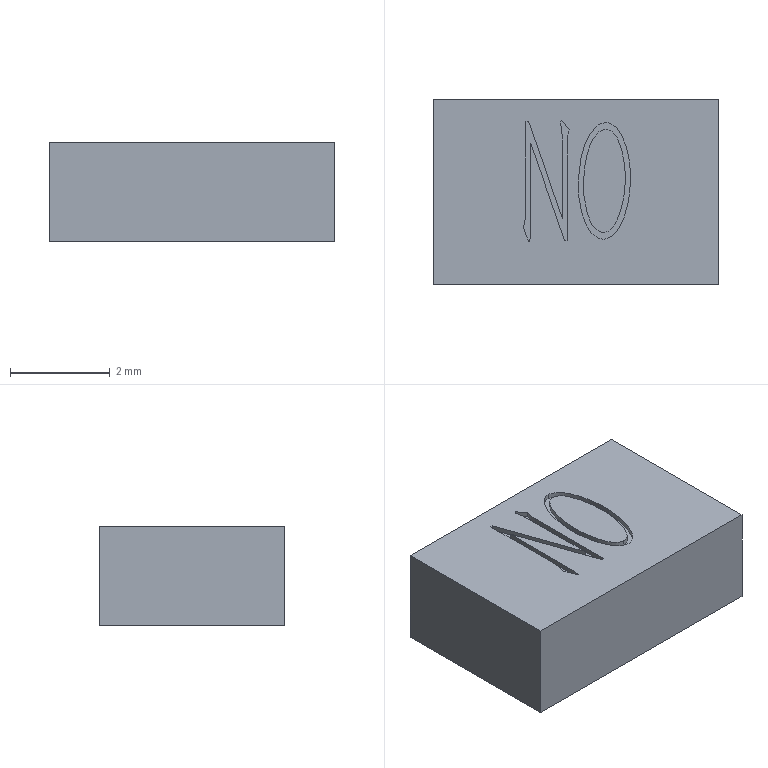Component | SolidWorks | Button1-1 | 1 solid | 33 faces | box 5.7 x 3.7 x 2 mm | volume 42 mm3 | plane 21 | spline 12
build123d program:
from build123d import *

# Parameters (mm, degrees)
SKETCH1_W           = 5.7
SKETCH1_H           = 3.7
BOSS_EXTRUDE1_DEPTH = 2
CUT_EXTRUDE1_DEPTH  = 0.1


with BuildPart() as part:
    # Sketch1 → Boss-Extrude1 (new body)
    with BuildSketch(Plane.XY):
        with Locations((2.85, 1.85)):
            Rectangle(SKETCH1_W, SKETCH1_H)
    extrude(amount=BOSS_EXTRUDE1_DEPTH)

    # Sketch2 → Cut-Extrude1 (cut)
    # profile 1 of 2: a face of its own
    with BuildSketch(Plane.XY.offset(2)):
        with BuildLine():
            Line((2.531, 3.25), (2.564, 3.282))
            Line((2.564, 3.282), (2.718, 3.092))
            add(Edge.make_bspline(
                [(2.718, 3.092), (2.715, 3.08), (2.708, 3.058), (2.697, 3.03), (2.691, 3.007), (2.687, 2.985), (2.683, 2.959), (2.679, 2.921), (2.676, 2.877), (2.675, 2.844), (2.675, 2.83)],
                knots=[0, 0, 0, 0, 1.084, 2.098, 2.644, 3.294, 4.083, 4.997, 6.707, 8, 8, 8, 8], degree=3))
            Line((2.675, 2.83), (2.675, 0.8842))
            Line((2.675, 0.8842), (2.621, 0.8842))
            Line((2.621, 0.8842), (1.945, 2.812))
            Line((1.945, 2.812), (1.945, 1.176))
            add(Edge.make_bspline(
                [(1.945, 1.176), (1.945, 1.162), (1.945, 1.133), (1.944, 1.087), (1.941, 1.036), (1.938, 0.9825), (1.935, 0.9341), (1.93, 0.8958), (1.927, 0.8739), (1.92, 0.8578), (1.905, 0.864), (1.894, 0.8769), (1.881, 0.9018), (1.874, 0.9221), (1.869, 0.9343)],
                knots=[0, 0, 0, 0, 1.182, 2.52, 4.031, 5.683, 7.211, 8.307, 8.99, 9.271, 9.606, 10.102, 10.868, 12, 12, 12, 12], degree=3))
            Line((1.869, 0.9343), (1.812, 1.096))
            add(Edge.make_bspline(
                [(1.812, 1.096), (1.808, 1.107), (1.802, 1.124), (1.798, 1.15), (1.804, 1.176), (1.811, 1.2), (1.818, 1.226), (1.824, 1.252), (1.829, 1.284), (1.835, 1.321), (1.842, 1.363), (1.845, 1.41), (1.848, 1.462), (1.848, 1.498), (1.848, 1.517)],
                knots=[0, 0, 0, 0, 0.9278, 1.561, 2.201, 3.116, 3.718, 4.47, 5.369, 6.414, 7.608, 8.945, 10.398, 12, 12, 12, 12], degree=3))
            Line((1.848, 1.517), (1.848, 3.257))
            Line((1.848, 3.257), (1.902, 3.257))
            Line((1.902, 3.257), (2.578, 1.323))
            Line((2.578, 1.323), (2.578, 2.826))
            add(Edge.make_bspline(
                [(2.578, 2.826), (2.578, 2.855), (2.577, 2.914), (2.573, 2.985), (2.57, 3.038), (2.567, 3.072), (2.564, 3.1), (2.561, 3.13), (2.556, 3.163), (2.549, 3.188), (2.545, 3.2)],
                knots=[0, 0, 0, 0, 1.88, 3.706, 4.546, 5.273, 5.876, 6.355, 7.192, 8, 8, 8, 8], degree=3))
            Line((2.545, 3.2), (2.531, 3.25))
        make_face()
    # profile 2 of 2: a face of its own
    with BuildSketch(Plane.XY.offset(2)):
        with BuildLine():
            add(Edge.make_bspline(
                [(2.899, 2.111), (2.901, 2.145), (2.906, 2.216), (2.919, 2.325), (2.935, 2.44), (2.956, 2.558), (2.982, 2.675), (3.017, 2.784), (3.059, 2.885), (3.108, 2.975), (3.16, 3.052), (3.211, 3.115), (3.258, 3.164), (3.304, 3.196), (3.349, 3.216), (3.389, 3.23), (3.427, 3.24), (3.452, 3.239), (3.464, 3.239)],
                knots=[0, 0, 0, 0, 1.218, 2.509, 3.869, 5.306, 6.733, 8.087, 9.358, 10.58, 11.689, 12.638, 13.421, 14.069, 14.629, 15.132, 15.587, 16, 16, 16, 16], degree=3))
            add(Edge.make_bspline(
                [(3.464, 3.239), (3.475, 3.237), (3.499, 3.233), (3.536, 3.219), (3.575, 3.199), (3.616, 3.173), (3.658, 3.139), (3.697, 3.096), (3.733, 3.044), (3.776, 2.964), (3.824, 2.853), (3.862, 2.736), (3.886, 2.636), (3.903, 2.557), (3.916, 2.474), (3.932, 2.357), (3.946, 2.209), (3.943, 2.09), (3.942, 2.031)],
                knots=[0, 0, 0, 0, 0.395, 0.8398, 1.348, 1.917, 2.536, 3.197, 3.916, 4.702, 6.363, 8.071, 8.963, 9.892, 10.869, 11.891, 13.955, 16, 16, 16, 16], degree=3))
            add(Edge.make_bspline(
                [(3.942, 2.031), (3.941, 2.009), (3.939, 1.963), (3.934, 1.892), (3.924, 1.816), (3.91, 1.71), (3.883, 1.573), (3.846, 1.438), (3.809, 1.332), (3.778, 1.257), (3.743, 1.185), (3.705, 1.119), (3.665, 1.06), (3.622, 1.01), (3.579, 0.9709), (3.534, 0.943), (3.491, 0.9241), (3.45, 0.9109), (3.413, 0.9044), (3.389, 0.9052), (3.378, 0.9055)],
                knots=[0, 0, 0, 0, 0.8813, 1.828, 2.828, 3.895, 6.098, 8.341, 9.452, 10.535, 11.578, 12.603, 13.56, 14.409, 15.182, 15.872, 16.496, 17.057, 17.549, 18, 18, 18, 18], degree=3))
            add(Edge.make_bspline(
                [(3.378, 0.9055), (3.366, 0.9069), (3.341, 0.9099), (3.303, 0.9224), (3.263, 0.9413), (3.221, 0.9668), (3.178, 1.001), (3.139, 1.047), (3.1, 1.102), (3.065, 1.167), (3.032, 1.24), (3.002, 1.319), (2.975, 1.401), (2.952, 1.488), (2.934, 1.575), (2.918, 1.661), (2.907, 1.745), (2.9, 1.825), (2.898, 1.902), (2.896, 1.975), (2.896, 2.044), (2.898, 2.089), (2.899, 2.111)],
                knots=[0, 0, 0, 0, 0.5105, 1.072, 1.705, 2.412, 3.189, 4.051, 5.012, 6.087, 7.247, 8.45, 9.695, 10.994, 12.293, 13.552, 14.755, 15.914, 17.024, 18.072, 19.066, 20, 20, 20, 20], degree=3))
        make_face()
        with BuildLine():
            add(Edge.make_bspline(
                [(3.004, 2.103), (3.003, 2.085), (3, 2.048), (3, 1.989), (3, 1.924), (3.004, 1.828), (3.016, 1.702), (3.038, 1.575), (3.062, 1.474), (3.084, 1.401), (3.107, 1.332), (3.133, 1.269), (3.161, 1.211), (3.192, 1.163), (3.223, 1.123), (3.257, 1.093), (3.29, 1.07), (3.322, 1.054), (3.352, 1.042), (3.372, 1.04), (3.381, 1.039)],
                knots=[0, 0, 0, 0, 0.7965, 1.68, 2.65, 3.709, 5.955, 8.313, 9.492, 10.627, 11.704, 12.746, 13.706, 14.554, 15.307, 15.977, 16.573, 17.107, 17.572, 18, 18, 18, 18], degree=3))
            add(Edge.make_bspline(
                [(3.381, 1.039), (3.391, 1.038), (3.411, 1.037), (3.442, 1.043), (3.475, 1.054), (3.509, 1.071), (3.544, 1.096), (3.577, 1.132), (3.61, 1.177), (3.643, 1.23), (3.675, 1.29), (3.703, 1.354), (3.729, 1.42), (3.757, 1.512), (3.788, 1.631), (3.813, 1.776), (3.83, 1.918), (3.84, 2.032), (3.841, 2.124), (3.839, 2.198), (3.835, 2.278), (3.83, 2.333), (3.827, 2.362)],
                knots=[0, 0, 0, 0, 0.3893, 0.8058, 1.253, 1.753, 2.311, 2.952, 3.695, 4.543, 5.455, 6.377, 7.318, 8.276, 10.228, 12.212, 14.137, 15.91, 16.802, 17.779, 18.849, 20, 20, 20, 20], degree=3))
            add(Edge.make_bspline(
                [(3.827, 2.362), (3.824, 2.388), (3.818, 2.439), (3.806, 2.512), (3.794, 2.58), (3.774, 2.664), (3.745, 2.765), (3.707, 2.862), (3.673, 2.934), (3.645, 2.982), (3.614, 3.02), (3.581, 3.051), (3.547, 3.073), (3.516, 3.091), (3.486, 3.102), (3.466, 3.105), (3.456, 3.106)],
                knots=[0, 0, 0, 0, 1.252, 2.433, 3.525, 4.55, 6.523, 8.527, 9.484, 10.352, 11.127, 11.838, 12.476, 13.043, 13.546, 14, 14, 14, 14], degree=3))
            add(Edge.make_bspline(
                [(3.456, 3.106), (3.447, 3.105), (3.428, 3.104), (3.397, 3.097), (3.365, 3.083), (3.33, 3.067), (3.292, 3.039), (3.254, 2.997), (3.214, 2.94), (3.171, 2.872), (3.131, 2.793), (3.097, 2.701), (3.068, 2.602), (3.048, 2.495), (3.031, 2.389), (3.019, 2.287), (3.008, 2.193), (3.005, 2.132), (3.004, 2.103)],
                knots=[0, 0, 0, 0, 0.3776, 0.8001, 1.267, 1.784, 2.394, 3.156, 4.087, 5.194, 6.426, 7.732, 9.139, 10.643, 12.142, 13.534, 14.82, 16, 16, 16, 16], degree=3))
        make_face(mode=Mode.SUBTRACT)
    extrude(amount=-CUT_EXTRUDE1_DEPTH, mode=Mode.SUBTRACT)


solid = part.part

# Placed as in the assembly
solid = solid.moved(Location((-75.506, -4.714, 277.152), (0, 0, 0)))